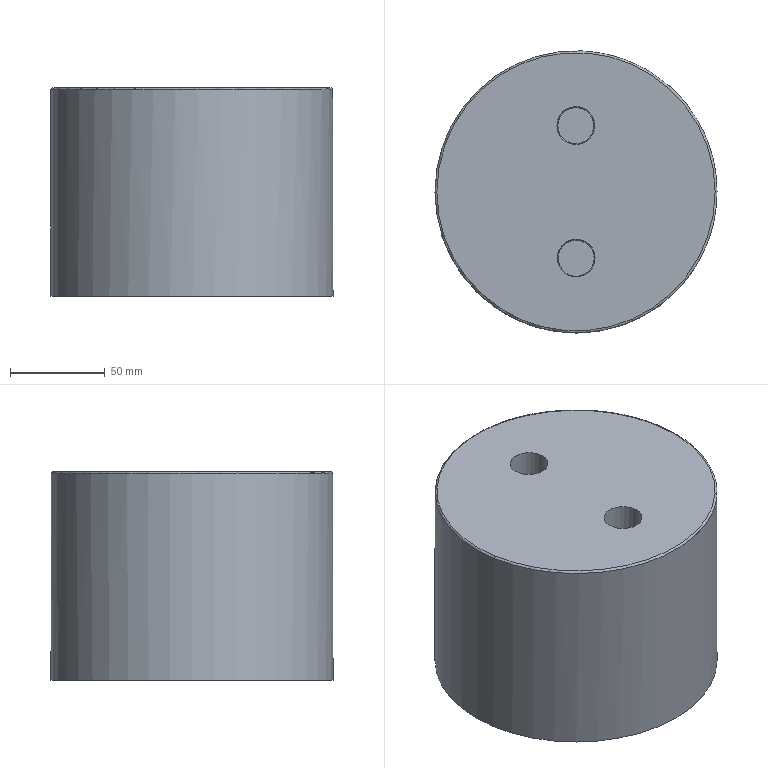Component | NX | A_PART_8 | 1 solid | 16 faces | box 149 x 149 x 110 mm | volume 1872912 mm3 | plane 8 | cylinder 5 | torus 3 | commonest cylinder face diameters 20 x2 149 x1 60 x1 15 x1
STEP:
#1=CARTESIAN_POINT('',(0.,0.,0.));
#2=DIRECTION('',(0.,0.,1.));
#3=DIRECTION('',(1.,0.,0.));
#4=AXIS2_PLACEMENT_3D('',#1,#2,#3);
#5=CARTESIAN_POINT('',(78.417,257.073,11.984));
#6=VERTEX_POINT('',#5);
#7=CARTESIAN_POINT('',(152.917,257.26,11.984));
#8=DIRECTION('',(0.,0.,-1.));
#9=DIRECTION('',(-1.,-0.0025,0.));
#10=AXIS2_PLACEMENT_3D('',#7,#8,#9);
#11=CIRCLE('',#10,74.5);
#12=CARTESIAN_POINT('',(152.917,257.26,12.984));
#13=DIRECTION('',(0.,0.,-1.));
#14=DIRECTION('',(-1.,-0.0025,0.));
#15=AXIS2_PLACEMENT_3D('',#12,#13,#14);
#16=CYLINDRICAL_SURFACE('',#15,74.5);
#17=CARTESIAN_POINT('',(0.,1.));
#18=DIRECTION('',(1.,0.));
#19=VECTOR('',#18,1.);
#20=LINE('',#17,#19);
#21=(GEOMETRIC_REPRESENTATION_CONTEXT(2)PARAMETRIC_REPRESENTATION_CONTEXT()REPRESENTATION_CONTEXT('',''));
#22=DEFINITIONAL_REPRESENTATION('',(#20),#21);
#23=PCURVE('',#16,#22);
#24=CARTESIAN_POINT('',(152.917,257.26,11.984));
#25=DIRECTION('',(0.,0.,-1.));
#26=DIRECTION('',(-1.,-0.0025,0.));
#27=AXIS2_PLACEMENT_3D('',#24,#25,#26);
#28=TOROIDAL_SURFACE('',#27,73.5,1.);
#29=CARTESIAN_POINT('',(0.,6.283));
#30=DIRECTION('',(1.,0.));
#31=VECTOR('',#30,1.);
#32=LINE('',#29,#31);
#33=(GEOMETRIC_REPRESENTATION_CONTEXT(2)PARAMETRIC_REPRESENTATION_CONTEXT()REPRESENTATION_CONTEXT('',''));
#34=DEFINITIONAL_REPRESENTATION('',(#32),#33);
#35=PCURVE('',#28,#34);
#36=SURFACE_CURVE('',#11,(#23,#35),.PCURVE_S1.);
#37=EDGE_CURVE('',#6,#6,#36,.T.);
#38=ORIENTED_EDGE('',*,*,#37,.T.);
#39=CARTESIAN_POINT('',(78.417,257.073,-97.016));
#40=VERTEX_POINT('',#39);
#41=CARTESIAN_POINT('',(78.417,257.073,11.984));
#42=CARTESIAN_POINT('',(78.417,257.073,-97.016));
#43=B_SPLINE_CURVE_WITH_KNOTS('',1,(#41,#42),.UNSPECIFIED.,.F.,.F.,(2,2),(1.,110.),.PIECEWISE_BEZIER_KNOTS.);
#44=CARTESIAN_POINT('',(6.283,0.));
#45=DIRECTION('',(0.,1.));
#46=VECTOR('',#45,1.);
#47=LINE('',#44,#46);
#48=(GEOMETRIC_REPRESENTATION_CONTEXT(2)PARAMETRIC_REPRESENTATION_CONTEXT()REPRESENTATION_CONTEXT('',''));
#49=DEFINITIONAL_REPRESENTATION('',(#47),#48);
#50=PCURVE('',#16,#49);
#51=CARTESIAN_POINT('',(0.,0.));
#52=DIRECTION('',(0.,1.));
#53=VECTOR('',#52,1.);
#54=LINE('',#51,#53);
#55=(GEOMETRIC_REPRESENTATION_CONTEXT(2)PARAMETRIC_REPRESENTATION_CONTEXT()REPRESENTATION_CONTEXT('',''));
#56=DEFINITIONAL_REPRESENTATION('',(#54),#55);
#57=PCURVE('',#16,#56);
#58=SEAM_CURVE('',#43,(#50,#57),.PCURVE_S1.);
#59=EDGE_CURVE('',#6,#40,#58,.T.);
#60=ORIENTED_EDGE('',*,*,#59,.T.);
#61=CARTESIAN_POINT('',(227.417,257.446,-97.016));
#62=VERTEX_POINT('',#61);
#63=CARTESIAN_POINT('',(152.917,257.26,-97.016));
#64=DIRECTION('',(0.,0.,-1.));
#65=DIRECTION('',(1.,0.0025,0.));
#66=AXIS2_PLACEMENT_3D('',#63,#64,#65);
#67=CIRCLE('',#66,74.5);
#68=CARTESIAN_POINT('',(3.142,110.));
#69=DIRECTION('',(1.,0.));
#70=VECTOR('',#69,1.);
#71=LINE('',#68,#70);
#72=(GEOMETRIC_REPRESENTATION_CONTEXT(2)PARAMETRIC_REPRESENTATION_CONTEXT()REPRESENTATION_CONTEXT('',''));
#73=DEFINITIONAL_REPRESENTATION('',(#71),#72);
#74=PCURVE('',#16,#73);
#75=CARTESIAN_POINT('',(152.917,257.26,-97.016));
#76=DIRECTION('',(0.,0.,-1.));
#77=DIRECTION('',(-1.,-0.0025,0.));
#78=AXIS2_PLACEMENT_3D('',#75,#76,#77);
#79=PLANE('',#78);
#80=CARTESIAN_POINT('',(0.,0.));
#81=DIRECTION('',(-1.,0.));
#82=AXIS2_PLACEMENT_2D('',#80,#81);
#83=CIRCLE('',#82,74.5);
#84=(GEOMETRIC_REPRESENTATION_CONTEXT(2)PARAMETRIC_REPRESENTATION_CONTEXT()REPRESENTATION_CONTEXT('',''));
#85=DEFINITIONAL_REPRESENTATION('',(#83),#84);
#86=PCURVE('',#79,#85);
#87=SURFACE_CURVE('',#67,(#74,#86),.PCURVE_S1.);
#88=EDGE_CURVE('',#62,#40,#87,.T.);
#89=ORIENTED_EDGE('',*,*,#88,.F.);
#90=CARTESIAN_POINT('',(152.917,257.26,-97.016));
#91=DIRECTION('',(0.,0.,-1.));
#92=DIRECTION('',(1.,0.0025,0.));
#93=AXIS2_PLACEMENT_3D('',#90,#91,#92);
#94=CIRCLE('',#93,74.5);
#95=CARTESIAN_POINT('',(-3.142,110.));
#96=DIRECTION('',(1.,0.));
#97=VECTOR('',#96,1.);
#98=LINE('',#95,#97);
#99=(GEOMETRIC_REPRESENTATION_CONTEXT(2)PARAMETRIC_REPRESENTATION_CONTEXT()REPRESENTATION_CONTEXT('',''));
#100=DEFINITIONAL_REPRESENTATION('',(#98),#99);
#101=PCURVE('',#16,#100);
#102=CARTESIAN_POINT('',(0.,0.));
#103=DIRECTION('',(-1.,0.));
#104=AXIS2_PLACEMENT_2D('',#102,#103);
#105=CIRCLE('',#104,74.5);
#106=(GEOMETRIC_REPRESENTATION_CONTEXT(2)PARAMETRIC_REPRESENTATION_CONTEXT()REPRESENTATION_CONTEXT('',''));
#107=DEFINITIONAL_REPRESENTATION('',(#105),#106);
#108=PCURVE('',#79,#107);
#109=SURFACE_CURVE('',#94,(#101,#108),.PCURVE_S1.);
#110=EDGE_CURVE('',#40,#62,#109,.T.);
#111=ORIENTED_EDGE('',*,*,#110,.F.);
#112=ORIENTED_EDGE('',*,*,#59,.F.);
#113=EDGE_LOOP('',(#38,#60,#89,#111,#112));
#114=FACE_BOUND('',#113,.T.);
#115=ADVANCED_FACE('',(#114),#16,.T.);
#116=CARTESIAN_POINT('',(163.004,222.285,12.984));
#117=VERTEX_POINT('',#116);
#118=CARTESIAN_POINT('',(153.004,222.26,12.984));
#119=DIRECTION('',(0.,0.,-1.));
#120=DIRECTION('',(1.,0.0025,0.));
#121=AXIS2_PLACEMENT_3D('',#118,#119,#120);
#122=CIRCLE('',#121,10.);
#123=CARTESIAN_POINT('',(152.917,257.26,12.984));
#124=DIRECTION('',(0.,0.,-1.));
#125=DIRECTION('',(-1.,-0.0025,0.));
#126=AXIS2_PLACEMENT_3D('',#123,#124,#125);
#127=PLANE('',#126);
#128=CARTESIAN_POINT('',(0.,-35.));
#129=DIRECTION('',(-1.,0.));
#130=AXIS2_PLACEMENT_2D('',#128,#129);
#131=CIRCLE('',#130,10.);
#132=(GEOMETRIC_REPRESENTATION_CONTEXT(2)PARAMETRIC_REPRESENTATION_CONTEXT()REPRESENTATION_CONTEXT('',''));
#133=DEFINITIONAL_REPRESENTATION('',(#131),#132);
#134=PCURVE('',#127,#133);
#135=CARTESIAN_POINT('',(153.004,222.26,-42.016));
#136=DIRECTION('',(0.,0.,1.));
#137=DIRECTION('',(1.,0.0025,0.));
#138=AXIS2_PLACEMENT_3D('',#135,#136,#137);
#139=CYLINDRICAL_SURFACE('',#138,10.);
#140=CARTESIAN_POINT('',(6.283,55.));
#141=DIRECTION('',(-1.,0.));
#142=VECTOR('',#141,1.);
#143=LINE('',#140,#142);
#144=(GEOMETRIC_REPRESENTATION_CONTEXT(2)PARAMETRIC_REPRESENTATION_CONTEXT()REPRESENTATION_CONTEXT('',''));
#145=DEFINITIONAL_REPRESENTATION('',(#143),#144);
#146=PCURVE('',#139,#145);
#147=SURFACE_CURVE('',#122,(#134,#146),.PCURVE_S1.);
#148=EDGE_CURVE('',#117,#117,#147,.T.);
#149=ORIENTED_EDGE('',*,*,#148,.T.);
#150=EDGE_LOOP('',(#149));
#151=FACE_BOUND('',#150,.T.);
#152=CARTESIAN_POINT('',(162.829,292.285,12.984));
#153=VERTEX_POINT('',#152);
#154=CARTESIAN_POINT('',(152.829,292.26,12.984));
#155=DIRECTION('',(0.,0.,-1.));
#156=DIRECTION('',(1.,0.0025,0.));
#157=AXIS2_PLACEMENT_3D('',#154,#155,#156);
#158=CIRCLE('',#157,10.);
#159=CARTESIAN_POINT('',(0.,35.));
#160=DIRECTION('',(-1.,0.));
#161=AXIS2_PLACEMENT_2D('',#159,#160);
#162=CIRCLE('',#161,10.);
#163=(GEOMETRIC_REPRESENTATION_CONTEXT(2)PARAMETRIC_REPRESENTATION_CONTEXT()REPRESENTATION_CONTEXT('',''));
#164=DEFINITIONAL_REPRESENTATION('',(#162),#163);
#165=PCURVE('',#127,#164);
#166=CARTESIAN_POINT('',(152.829,292.26,-42.016));
#167=DIRECTION('',(0.,0.,1.));
#168=DIRECTION('',(1.,0.0025,0.));
#169=AXIS2_PLACEMENT_3D('',#166,#167,#168);
#170=CYLINDRICAL_SURFACE('',#169,10.);
#171=CARTESIAN_POINT('',(6.283,55.));
#172=DIRECTION('',(-1.,0.));
#173=VECTOR('',#172,1.);
#174=LINE('',#171,#173);
#175=(GEOMETRIC_REPRESENTATION_CONTEXT(2)PARAMETRIC_REPRESENTATION_CONTEXT()REPRESENTATION_CONTEXT('',''));
#176=DEFINITIONAL_REPRESENTATION('',(#174),#175);
#177=PCURVE('',#170,#176);
#178=SURFACE_CURVE('',#158,(#165,#177),.PCURVE_S1.);
#179=EDGE_CURVE('',#153,#153,#178,.T.);
#180=ORIENTED_EDGE('',*,*,#179,.T.);
#181=EDGE_LOOP('',(#180));
#182=FACE_BOUND('',#181,.T.);
#183=CARTESIAN_POINT('',(79.417,257.076,12.984));
#184=VERTEX_POINT('',#183);
#185=CARTESIAN_POINT('',(152.917,257.26,12.984));
#186=DIRECTION('',(0.,0.,1.));
#187=DIRECTION('',(-1.,-0.0025,0.));
#188=AXIS2_PLACEMENT_3D('',#185,#186,#187);
#189=CIRCLE('',#188,73.5);
#190=CARTESIAN_POINT('',(73.5,-0.));
#191=CARTESIAN_POINT('',(73.5,-127.306));
#192=CARTESIAN_POINT('',(-36.75,-63.653));
#193=CARTESIAN_POINT('',(-147.,0.));
#194=CARTESIAN_POINT('',(-36.75,63.653));
#195=CARTESIAN_POINT('',(73.5,127.306));
#196=CARTESIAN_POINT('',(73.5,-0.));
#197=(BOUNDED_CURVE()B_SPLINE_CURVE(2,(#190,#191,#192,#193,#194,#195,#196),.UNSPECIFIED.,.T.,.F.)B_SPLINE_CURVE_WITH_KNOTS((1,2,2,2,2,1),(-2.094,0.,2.094,4.189,6.283,8.378),.UNSPECIFIED.)CURVE()GEOMETRIC_REPRESENTATION_ITEM()RATIONAL_B_SPLINE_CURVE((1.,0.5,1.,0.5,1.,0.5,1.))REPRESENTATION_ITEM(''));
#198=(GEOMETRIC_REPRESENTATION_CONTEXT(2)PARAMETRIC_REPRESENTATION_CONTEXT()REPRESENTATION_CONTEXT('',''));
#199=DEFINITIONAL_REPRESENTATION('',(#197),#198);
#200=PCURVE('',#127,#199);
#201=CARTESIAN_POINT('',(6.283,4.712));
#202=DIRECTION('',(-1.,0.));
#203=VECTOR('',#202,1.);
#204=LINE('',#201,#203);
#205=(GEOMETRIC_REPRESENTATION_CONTEXT(2)PARAMETRIC_REPRESENTATION_CONTEXT()REPRESENTATION_CONTEXT('',''));
#206=DEFINITIONAL_REPRESENTATION('',(#204),#205);
#207=PCURVE('',#28,#206);
#208=SURFACE_CURVE('',#189,(#200,#207),.PCURVE_S1.);
#209=EDGE_CURVE('',#184,#184,#208,.T.);
#210=ORIENTED_EDGE('',*,*,#209,.T.);
#211=EDGE_LOOP('',(#210));
#212=FACE_BOUND('',#211,.T.);
#213=ADVANCED_FACE('',(#151,#182,#212),#127,.F.);
#214=CARTESIAN_POINT('',(182.917,257.335,-97.016));
#215=VERTEX_POINT('',#214);
#216=CARTESIAN_POINT('',(152.917,257.26,-97.016));
#217=DIRECTION('',(0.,0.,-1.));
#218=DIRECTION('',(1.,0.0025,0.));
#219=AXIS2_PLACEMENT_3D('',#216,#217,#218);
#220=CIRCLE('',#219,30.);
#221=CARTESIAN_POINT('',(0.,0.));
#222=DIRECTION('',(-1.,0.));
#223=AXIS2_PLACEMENT_2D('',#221,#222);
#224=CIRCLE('',#223,30.);
#225=(GEOMETRIC_REPRESENTATION_CONTEXT(2)PARAMETRIC_REPRESENTATION_CONTEXT()REPRESENTATION_CONTEXT('',''));
#226=DEFINITIONAL_REPRESENTATION('',(#224),#225);
#227=PCURVE('',#79,#226);
#228=CARTESIAN_POINT('',(152.917,257.26,-95.016));
#229=DIRECTION('',(0.,0.,-1.));
#230=DIRECTION('',(-1.,-0.0025,0.));
#231=AXIS2_PLACEMENT_3D('',#228,#229,#230);
#232=CYLINDRICAL_SURFACE('',#231,30.);
#233=CARTESIAN_POINT('',(3.142,2.));
#234=DIRECTION('',(1.,0.));
#235=VECTOR('',#234,1.);
#236=LINE('',#233,#235);
#237=(GEOMETRIC_REPRESENTATION_CONTEXT(2)PARAMETRIC_REPRESENTATION_CONTEXT()REPRESENTATION_CONTEXT('',''));
#238=DEFINITIONAL_REPRESENTATION('',(#236),#237);
#239=PCURVE('',#232,#238);
#240=SURFACE_CURVE('',#220,(#227,#239),.PCURVE_S1.);
#241=EDGE_CURVE('',#215,#215,#240,.T.);
#242=ORIENTED_EDGE('',*,*,#241,.F.);
#243=EDGE_LOOP('',(#242));
#244=FACE_BOUND('',#243,.T.);
#245=ORIENTED_EDGE('',*,*,#88,.T.);
#246=ORIENTED_EDGE('',*,*,#110,.T.);
#247=EDGE_LOOP('',(#245,#246));
#248=FACE_BOUND('',#247,.T.);
#249=ADVANCED_FACE('',(#244,#248),#79,.T.);
#250=ORIENTED_EDGE('',*,*,#209,.F.);
#251=CARTESIAN_POINT('',(79.417,257.076,12.984));
#252=CARTESIAN_POINT('',(79.15,257.075,12.984));
#253=CARTESIAN_POINT('',(78.889,257.075,12.899));
#254=CARTESIAN_POINT('',(78.665,257.074,12.736));
#255=CARTESIAN_POINT('',(78.502,257.074,12.511));
#256=CARTESIAN_POINT('',(78.417,257.073,12.251));
#257=CARTESIAN_POINT('',(78.417,257.073,11.984));
#258=(BOUNDED_CURVE()B_SPLINE_CURVE(6,(#251,#252,#253,#254,#255,#256,#257),.UNSPECIFIED.,.F.,.F.)B_SPLINE_CURVE_WITH_KNOTS((7,7),(4.712,6.283),.PIECEWISE_BEZIER_KNOTS.)CURVE()GEOMETRIC_REPRESENTATION_ITEM()RATIONAL_B_SPLINE_CURVE((1.031,1.01,0.9979,0.994,0.9979,1.01,1.031))REPRESENTATION_ITEM(''));
#259=CARTESIAN_POINT('',(6.283,0.));
#260=DIRECTION('',(0.,1.));
#261=VECTOR('',#260,1.);
#262=LINE('',#259,#261);
#263=(GEOMETRIC_REPRESENTATION_CONTEXT(2)PARAMETRIC_REPRESENTATION_CONTEXT()REPRESENTATION_CONTEXT('',''));
#264=DEFINITIONAL_REPRESENTATION('',(#262),#263);
#265=PCURVE('',#28,#264);
#266=CARTESIAN_POINT('',(0.,0.));
#267=DIRECTION('',(0.,1.));
#268=VECTOR('',#267,1.);
#269=LINE('',#266,#268);
#270=(GEOMETRIC_REPRESENTATION_CONTEXT(2)PARAMETRIC_REPRESENTATION_CONTEXT()REPRESENTATION_CONTEXT('',''));
#271=DEFINITIONAL_REPRESENTATION('',(#269),#270);
#272=PCURVE('',#28,#271);
#273=SEAM_CURVE('',#258,(#265,#272),.PCURVE_S1.);
#274=EDGE_CURVE('',#184,#6,#273,.T.);
#275=ORIENTED_EDGE('',*,*,#274,.T.);
#276=ORIENTED_EDGE('',*,*,#37,.F.);
#277=ORIENTED_EDGE('',*,*,#274,.F.);
#278=EDGE_LOOP('',(#250,#275,#276,#277));
#279=FACE_BOUND('',#278,.T.);
#280=ADVANCED_FACE('',(#279),#28,.T.);
#281=CARTESIAN_POINT('',(162.829,292.285,-41.516));
#282=VERTEX_POINT('',#281);
#283=CARTESIAN_POINT('',(142.829,292.235,-41.516));
#284=VERTEX_POINT('',#283);
#285=CARTESIAN_POINT('',(152.829,292.26,-41.516));
#286=DIRECTION('',(0.,0.,-1.));
#287=DIRECTION('',(-1.,-0.0025,0.));
#288=AXIS2_PLACEMENT_3D('',#285,#286,#287);
#289=CIRCLE('',#288,10.);
#290=CARTESIAN_POINT('',(9.425,0.5));
#291=DIRECTION('',(-1.,0.));
#292=VECTOR('',#291,1.);
#293=LINE('',#290,#292);
#294=(GEOMETRIC_REPRESENTATION_CONTEXT(2)PARAMETRIC_REPRESENTATION_CONTEXT()REPRESENTATION_CONTEXT('',''));
#295=DEFINITIONAL_REPRESENTATION('',(#293),#294);
#296=PCURVE('',#170,#295);
#297=CARTESIAN_POINT('',(152.829,292.26,-41.516));
#298=DIRECTION('',(0.,0.,-1.));
#299=DIRECTION('',(-1.,-0.0025,0.));
#300=AXIS2_PLACEMENT_3D('',#297,#298,#299);
#301=TOROIDAL_SURFACE('',#300,9.5,0.5);
#302=CARTESIAN_POINT('',(0.,6.283));
#303=DIRECTION('',(1.,0.));
#304=VECTOR('',#303,1.);
#305=LINE('',#302,#304);
#306=(GEOMETRIC_REPRESENTATION_CONTEXT(2)PARAMETRIC_REPRESENTATION_CONTEXT()REPRESENTATION_CONTEXT('',''));
#307=DEFINITIONAL_REPRESENTATION('',(#305),#306);
#308=PCURVE('',#301,#307);
#309=SURFACE_CURVE('',#289,(#296,#308),.PCURVE_S1.);
#310=EDGE_CURVE('',#282,#284,#309,.T.);
#311=ORIENTED_EDGE('',*,*,#310,.F.);
#312=CARTESIAN_POINT('',(162.829,292.285,-41.516));
#313=CARTESIAN_POINT('',(162.829,292.285,12.984));
#314=B_SPLINE_CURVE_WITH_KNOTS('',1,(#312,#313),.UNSPECIFIED.,.F.,.F.,(2,2),(0.5,55.),.PIECEWISE_BEZIER_KNOTS.);
#315=CARTESIAN_POINT('',(6.283,0.));
#316=DIRECTION('',(0.,1.));
#317=VECTOR('',#316,1.);
#318=LINE('',#315,#317);
#319=(GEOMETRIC_REPRESENTATION_CONTEXT(2)PARAMETRIC_REPRESENTATION_CONTEXT()REPRESENTATION_CONTEXT('',''));
#320=DEFINITIONAL_REPRESENTATION('',(#318),#319);
#321=PCURVE('',#170,#320);
#322=CARTESIAN_POINT('',(0.,0.));
#323=DIRECTION('',(0.,1.));
#324=VECTOR('',#323,1.);
#325=LINE('',#322,#324);
#326=(GEOMETRIC_REPRESENTATION_CONTEXT(2)PARAMETRIC_REPRESENTATION_CONTEXT()REPRESENTATION_CONTEXT('',''));
#327=DEFINITIONAL_REPRESENTATION('',(#325),#326);
#328=PCURVE('',#170,#327);
#329=SEAM_CURVE('',#314,(#321,#328),.PCURVE_S1.);
#330=EDGE_CURVE('',#282,#153,#329,.T.);
#331=ORIENTED_EDGE('',*,*,#330,.T.);
#332=ORIENTED_EDGE('',*,*,#179,.T.);
#333=ORIENTED_EDGE('',*,*,#330,.F.);
#334=CARTESIAN_POINT('',(152.829,292.26,-41.516));
#335=DIRECTION('',(0.,0.,-1.));
#336=DIRECTION('',(-1.,-0.0025,0.));
#337=AXIS2_PLACEMENT_3D('',#334,#335,#336);
#338=CIRCLE('',#337,10.);
#339=CARTESIAN_POINT('',(3.142,0.5));
#340=DIRECTION('',(-1.,0.));
#341=VECTOR('',#340,1.);
#342=LINE('',#339,#341);
#343=(GEOMETRIC_REPRESENTATION_CONTEXT(2)PARAMETRIC_REPRESENTATION_CONTEXT()REPRESENTATION_CONTEXT('',''));
#344=DEFINITIONAL_REPRESENTATION('',(#342),#343);
#345=PCURVE('',#170,#344);
#346=CARTESIAN_POINT('',(0.,6.283));
#347=DIRECTION('',(1.,0.));
#348=VECTOR('',#347,1.);
#349=LINE('',#346,#348);
#350=(GEOMETRIC_REPRESENTATION_CONTEXT(2)PARAMETRIC_REPRESENTATION_CONTEXT()REPRESENTATION_CONTEXT('',''));
#351=DEFINITIONAL_REPRESENTATION('',(#349),#350);
#352=PCURVE('',#301,#351);
#353=SURFACE_CURVE('',#338,(#345,#352),.PCURVE_S1.);
#354=EDGE_CURVE('',#284,#282,#353,.T.);
#355=ORIENTED_EDGE('',*,*,#354,.F.);
#356=EDGE_LOOP('',(#311,#331,#332,#333,#355));
#357=FACE_BOUND('',#356,.F.);
#358=ADVANCED_FACE('',(#357),#170,.F.);
#359=CARTESIAN_POINT('',(143.329,292.236,-42.016));
#360=VERTEX_POINT('',#359);
#361=CARTESIAN_POINT('',(152.829,292.26,-42.016));
#362=DIRECTION('',(0.,0.,1.));
#363=DIRECTION('',(-1.,-0.0025,0.));
#364=AXIS2_PLACEMENT_3D('',#361,#362,#363);
#365=CIRCLE('',#364,9.5);
#366=CARTESIAN_POINT('',(152.829,292.26,-42.016));
#367=DIRECTION('',(0.,0.,-1.));
#368=DIRECTION('',(-1.,-0.0025,0.));
#369=AXIS2_PLACEMENT_3D('',#366,#367,#368);
#370=PLANE('',#369);
#371=CARTESIAN_POINT('',(9.5,-0.));
#372=CARTESIAN_POINT('',(9.5,-16.454));
#373=CARTESIAN_POINT('',(-4.75,-8.227));
#374=CARTESIAN_POINT('',(-19.,0.));
#375=CARTESIAN_POINT('',(-4.75,8.227));
#376=CARTESIAN_POINT('',(9.5,16.454));
#377=CARTESIAN_POINT('',(9.5,-0.));
#378=(BOUNDED_CURVE()B_SPLINE_CURVE(2,(#371,#372,#373,#374,#375,#376,#377),.UNSPECIFIED.,.T.,.F.)B_SPLINE_CURVE_WITH_KNOTS((1,2,2,2,2,1),(-2.094,0.,2.094,4.189,6.283,8.378),.UNSPECIFIED.)CURVE()GEOMETRIC_REPRESENTATION_ITEM()RATIONAL_B_SPLINE_CURVE((1.,0.5,1.,0.5,1.,0.5,1.))REPRESENTATION_ITEM(''));
#379=(GEOMETRIC_REPRESENTATION_CONTEXT(2)PARAMETRIC_REPRESENTATION_CONTEXT()REPRESENTATION_CONTEXT('',''));
#380=DEFINITIONAL_REPRESENTATION('',(#378),#379);
#381=PCURVE('',#370,#380);
#382=CARTESIAN_POINT('',(6.283,7.854));
#383=DIRECTION('',(-1.,0.));
#384=VECTOR('',#383,1.);
#385=LINE('',#382,#384);
#386=(GEOMETRIC_REPRESENTATION_CONTEXT(2)PARAMETRIC_REPRESENTATION_CONTEXT()REPRESENTATION_CONTEXT('',''));
#387=DEFINITIONAL_REPRESENTATION('',(#385),#386);
#388=PCURVE('',#301,#387);
#389=SURFACE_CURVE('',#365,(#381,#388),.PCURVE_S1.);
#390=EDGE_CURVE('',#360,#360,#389,.T.);
#391=ORIENTED_EDGE('',*,*,#390,.T.);
#392=EDGE_LOOP('',(#391));
#393=FACE_BOUND('',#392,.T.);
#394=ADVANCED_FACE('',(#393),#370,.F.);
#395=CARTESIAN_POINT('',(163.004,222.285,-41.516));
#396=VERTEX_POINT('',#395);
#397=CARTESIAN_POINT('',(143.004,222.235,-41.516));
#398=VERTEX_POINT('',#397);
#399=CARTESIAN_POINT('',(153.004,222.26,-41.516));
#400=DIRECTION('',(0.,0.,-1.));
#401=DIRECTION('',(-1.,-0.0025,0.));
#402=AXIS2_PLACEMENT_3D('',#399,#400,#401);
#403=CIRCLE('',#402,10.);
#404=CARTESIAN_POINT('',(9.425,0.5));
#405=DIRECTION('',(-1.,0.));
#406=VECTOR('',#405,1.);
#407=LINE('',#404,#406);
#408=(GEOMETRIC_REPRESENTATION_CONTEXT(2)PARAMETRIC_REPRESENTATION_CONTEXT()REPRESENTATION_CONTEXT('',''));
#409=DEFINITIONAL_REPRESENTATION('',(#407),#408);
#410=PCURVE('',#139,#409);
#411=CARTESIAN_POINT('',(153.004,222.26,-41.516));
#412=DIRECTION('',(0.,0.,-1.));
#413=DIRECTION('',(-1.,-0.0025,0.));
#414=AXIS2_PLACEMENT_3D('',#411,#412,#413);
#415=TOROIDAL_SURFACE('',#414,9.5,0.5);
#416=CARTESIAN_POINT('',(-0.,6.283));
#417=DIRECTION('',(1.,0.));
#418=VECTOR('',#417,1.);
#419=LINE('',#416,#418);
#420=(GEOMETRIC_REPRESENTATION_CONTEXT(2)PARAMETRIC_REPRESENTATION_CONTEXT()REPRESENTATION_CONTEXT('',''));
#421=DEFINITIONAL_REPRESENTATION('',(#419),#420);
#422=PCURVE('',#415,#421);
#423=SURFACE_CURVE('',#403,(#410,#422),.PCURVE_S1.);
#424=EDGE_CURVE('',#396,#398,#423,.T.);
#425=ORIENTED_EDGE('',*,*,#424,.F.);
#426=CARTESIAN_POINT('',(163.004,222.285,-41.516));
#427=CARTESIAN_POINT('',(163.004,222.285,12.984));
#428=B_SPLINE_CURVE_WITH_KNOTS('',1,(#426,#427),.UNSPECIFIED.,.F.,.F.,(2,2),(0.5,55.),.PIECEWISE_BEZIER_KNOTS.);
#429=CARTESIAN_POINT('',(6.283,0.));
#430=DIRECTION('',(0.,1.));
#431=VECTOR('',#430,1.);
#432=LINE('',#429,#431);
#433=(GEOMETRIC_REPRESENTATION_CONTEXT(2)PARAMETRIC_REPRESENTATION_CONTEXT()REPRESENTATION_CONTEXT('',''));
#434=DEFINITIONAL_REPRESENTATION('',(#432),#433);
#435=PCURVE('',#139,#434);
#436=CARTESIAN_POINT('',(0.,0.));
#437=DIRECTION('',(0.,1.));
#438=VECTOR('',#437,1.);
#439=LINE('',#436,#438);
#440=(GEOMETRIC_REPRESENTATION_CONTEXT(2)PARAMETRIC_REPRESENTATION_CONTEXT()REPRESENTATION_CONTEXT('',''));
#441=DEFINITIONAL_REPRESENTATION('',(#439),#440);
#442=PCURVE('',#139,#441);
#443=SEAM_CURVE('',#428,(#435,#442),.PCURVE_S1.);
#444=EDGE_CURVE('',#396,#117,#443,.T.);
#445=ORIENTED_EDGE('',*,*,#444,.T.);
#446=ORIENTED_EDGE('',*,*,#148,.T.);
#447=ORIENTED_EDGE('',*,*,#444,.F.);
#448=CARTESIAN_POINT('',(153.004,222.26,-41.516));
#449=DIRECTION('',(0.,0.,-1.));
#450=DIRECTION('',(-1.,-0.0025,0.));
#451=AXIS2_PLACEMENT_3D('',#448,#449,#450);
#452=CIRCLE('',#451,10.);
#453=CARTESIAN_POINT('',(3.142,0.5));
#454=DIRECTION('',(-1.,0.));
#455=VECTOR('',#454,1.);
#456=LINE('',#453,#455);
#457=(GEOMETRIC_REPRESENTATION_CONTEXT(2)PARAMETRIC_REPRESENTATION_CONTEXT()REPRESENTATION_CONTEXT('',''));
#458=DEFINITIONAL_REPRESENTATION('',(#456),#457);
#459=PCURVE('',#139,#458);
#460=CARTESIAN_POINT('',(0.,6.283));
#461=DIRECTION('',(1.,0.));
#462=VECTOR('',#461,1.);
#463=LINE('',#460,#462);
#464=(GEOMETRIC_REPRESENTATION_CONTEXT(2)PARAMETRIC_REPRESENTATION_CONTEXT()REPRESENTATION_CONTEXT('',''));
#465=DEFINITIONAL_REPRESENTATION('',(#463),#464);
#466=PCURVE('',#415,#465);
#467=SURFACE_CURVE('',#452,(#459,#466),.PCURVE_S1.);
#468=EDGE_CURVE('',#398,#396,#467,.T.);
#469=ORIENTED_EDGE('',*,*,#468,.F.);
#470=EDGE_LOOP('',(#425,#445,#446,#447,#469));
#471=FACE_BOUND('',#470,.F.);
#472=ADVANCED_FACE('',(#471),#139,.F.);
#473=CARTESIAN_POINT('',(143.504,222.236,-42.016));
#474=VERTEX_POINT('',#473);
#475=CARTESIAN_POINT('',(153.004,222.26,-42.016));
#476=DIRECTION('',(0.,0.,1.));
#477=DIRECTION('',(-1.,-0.0025,0.));
#478=AXIS2_PLACEMENT_3D('',#475,#476,#477);
#479=CIRCLE('',#478,9.5);
#480=CARTESIAN_POINT('',(153.004,222.26,-42.016));
#481=DIRECTION('',(0.,0.,-1.));
#482=DIRECTION('',(-1.,-0.0025,0.));
#483=AXIS2_PLACEMENT_3D('',#480,#481,#482);
#484=PLANE('',#483);
#485=CARTESIAN_POINT('',(9.5,-0.));
#486=CARTESIAN_POINT('',(9.5,-16.454));
#487=CARTESIAN_POINT('',(-4.75,-8.227));
#488=CARTESIAN_POINT('',(-19.,0.));
#489=CARTESIAN_POINT('',(-4.75,8.227));
#490=CARTESIAN_POINT('',(9.5,16.454));
#491=CARTESIAN_POINT('',(9.5,-0.));
#492=(BOUNDED_CURVE()B_SPLINE_CURVE(2,(#485,#486,#487,#488,#489,#490,#491),.UNSPECIFIED.,.T.,.F.)B_SPLINE_CURVE_WITH_KNOTS((1,2,2,2,2,1),(-2.094,0.,2.094,4.189,6.283,8.378),.UNSPECIFIED.)CURVE()GEOMETRIC_REPRESENTATION_ITEM()RATIONAL_B_SPLINE_CURVE((1.,0.5,1.,0.5,1.,0.5,1.))REPRESENTATION_ITEM(''));
#493=(GEOMETRIC_REPRESENTATION_CONTEXT(2)PARAMETRIC_REPRESENTATION_CONTEXT()REPRESENTATION_CONTEXT('',''));
#494=DEFINITIONAL_REPRESENTATION('',(#492),#493);
#495=PCURVE('',#484,#494);
#496=CARTESIAN_POINT('',(6.283,7.854));
#497=DIRECTION('',(-1.,0.));
#498=VECTOR('',#497,1.);
#499=LINE('',#496,#498);
#500=(GEOMETRIC_REPRESENTATION_CONTEXT(2)PARAMETRIC_REPRESENTATION_CONTEXT()REPRESENTATION_CONTEXT('',''));
#501=DEFINITIONAL_REPRESENTATION('',(#499),#500);
#502=PCURVE('',#415,#501);
#503=SURFACE_CURVE('',#479,(#495,#502),.PCURVE_S1.);
#504=EDGE_CURVE('',#474,#474,#503,.T.);
#505=ORIENTED_EDGE('',*,*,#504,.T.);
#506=EDGE_LOOP('',(#505));
#507=FACE_BOUND('',#506,.T.);
#508=ADVANCED_FACE('',(#507),#484,.F.);
#509=ORIENTED_EDGE('',*,*,#310,.T.);
#510=CARTESIAN_POINT('',(142.829,292.235,-41.516));
#511=CARTESIAN_POINT('',(142.829,292.235,-41.65));
#512=CARTESIAN_POINT('',(142.872,292.235,-41.78));
#513=CARTESIAN_POINT('',(142.953,292.235,-41.892));
#514=CARTESIAN_POINT('',(143.065,292.235,-41.974));
#515=CARTESIAN_POINT('',(143.196,292.235,-42.016));
#516=CARTESIAN_POINT('',(143.329,292.236,-42.016));
#517=(BOUNDED_CURVE()B_SPLINE_CURVE(6,(#510,#511,#512,#513,#514,#515,#516),.UNSPECIFIED.,.F.,.F.)B_SPLINE_CURVE_WITH_KNOTS((7,7),(0.,1.571),.PIECEWISE_BEZIER_KNOTS.)CURVE()GEOMETRIC_REPRESENTATION_ITEM()RATIONAL_B_SPLINE_CURVE((1.031,1.01,0.9979,0.994,0.9979,1.01,1.031))REPRESENTATION_ITEM(''));
#518=CARTESIAN_POINT('',(6.283,6.283));
#519=DIRECTION('',(0.,1.));
#520=VECTOR('',#519,1.);
#521=LINE('',#518,#520);
#522=(GEOMETRIC_REPRESENTATION_CONTEXT(2)PARAMETRIC_REPRESENTATION_CONTEXT()REPRESENTATION_CONTEXT('',''));
#523=DEFINITIONAL_REPRESENTATION('',(#521),#522);
#524=PCURVE('',#301,#523);
#525=CARTESIAN_POINT('',(0.,6.283));
#526=DIRECTION('',(0.,1.));
#527=VECTOR('',#526,1.);
#528=LINE('',#525,#527);
#529=(GEOMETRIC_REPRESENTATION_CONTEXT(2)PARAMETRIC_REPRESENTATION_CONTEXT()REPRESENTATION_CONTEXT('',''));
#530=DEFINITIONAL_REPRESENTATION('',(#528),#529);
#531=PCURVE('',#301,#530);
#532=SEAM_CURVE('',#517,(#524,#531),.PCURVE_S1.);
#533=EDGE_CURVE('',#284,#360,#532,.T.);
#534=ORIENTED_EDGE('',*,*,#533,.T.);
#535=ORIENTED_EDGE('',*,*,#390,.T.);
#536=ORIENTED_EDGE('',*,*,#533,.F.);
#537=ORIENTED_EDGE('',*,*,#354,.T.);
#538=EDGE_LOOP('',(#509,#534,#535,#536,#537));
#539=FACE_BOUND('',#538,.F.);
#540=ADVANCED_FACE('',(#539),#301,.F.);
#541=ORIENTED_EDGE('',*,*,#424,.T.);
#542=CARTESIAN_POINT('',(143.004,222.235,-41.516));
#543=CARTESIAN_POINT('',(143.004,222.235,-41.65));
#544=CARTESIAN_POINT('',(143.047,222.235,-41.78));
#545=CARTESIAN_POINT('',(143.128,222.235,-41.892));
#546=CARTESIAN_POINT('',(143.24,222.235,-41.974));
#547=CARTESIAN_POINT('',(143.371,222.236,-42.016));
#548=CARTESIAN_POINT('',(143.504,222.236,-42.016));
#549=(BOUNDED_CURVE()B_SPLINE_CURVE(6,(#542,#543,#544,#545,#546,#547,#548),.UNSPECIFIED.,.F.,.F.)B_SPLINE_CURVE_WITH_KNOTS((7,7),(0.,1.571),.PIECEWISE_BEZIER_KNOTS.)CURVE()GEOMETRIC_REPRESENTATION_ITEM()RATIONAL_B_SPLINE_CURVE((1.031,1.01,0.9979,0.994,0.9979,1.01,1.031))REPRESENTATION_ITEM(''));
#550=CARTESIAN_POINT('',(6.283,6.283));
#551=DIRECTION('',(0.,1.));
#552=VECTOR('',#551,1.);
#553=LINE('',#550,#552);
#554=(GEOMETRIC_REPRESENTATION_CONTEXT(2)PARAMETRIC_REPRESENTATION_CONTEXT()REPRESENTATION_CONTEXT('',''));
#555=DEFINITIONAL_REPRESENTATION('',(#553),#554);
#556=PCURVE('',#415,#555);
#557=CARTESIAN_POINT('',(-0.,6.283));
#558=DIRECTION('',(0.,1.));
#559=VECTOR('',#558,1.);
#560=LINE('',#557,#559);
#561=(GEOMETRIC_REPRESENTATION_CONTEXT(2)PARAMETRIC_REPRESENTATION_CONTEXT()REPRESENTATION_CONTEXT('',''));
#562=DEFINITIONAL_REPRESENTATION('',(#560),#561);
#563=PCURVE('',#415,#562);
#564=SEAM_CURVE('',#549,(#556,#563),.PCURVE_S1.);
#565=EDGE_CURVE('',#398,#474,#564,.T.);
#566=ORIENTED_EDGE('',*,*,#565,.T.);
#567=ORIENTED_EDGE('',*,*,#504,.T.);
#568=ORIENTED_EDGE('',*,*,#565,.F.);
#569=ORIENTED_EDGE('',*,*,#468,.T.);
#570=EDGE_LOOP('',(#541,#566,#567,#568,#569));
#571=FACE_BOUND('',#570,.F.);
#572=ADVANCED_FACE('',(#571),#415,.F.);
#573=CARTESIAN_POINT('',(182.917,257.335,-95.016));
#574=VERTEX_POINT('',#573);
#575=CARTESIAN_POINT('',(152.917,257.26,-95.016));
#576=DIRECTION('',(0.,0.,1.));
#577=DIRECTION('',(1.,0.0025,0.));
#578=AXIS2_PLACEMENT_3D('',#575,#576,#577);
#579=CIRCLE('',#578,30.);
#580=CARTESIAN_POINT('',(9.425,0.));
#581=DIRECTION('',(-1.,0.));
#582=VECTOR('',#581,1.);
#583=LINE('',#580,#582);
#584=(GEOMETRIC_REPRESENTATION_CONTEXT(2)PARAMETRIC_REPRESENTATION_CONTEXT()REPRESENTATION_CONTEXT('',''));
#585=DEFINITIONAL_REPRESENTATION('',(#583),#584);
#586=PCURVE('',#232,#585);
#587=CARTESIAN_POINT('',(152.917,257.26,-95.016));
#588=DIRECTION('',(0.,0.,-1.));
#589=DIRECTION('',(-1.,-0.0025,0.));
#590=AXIS2_PLACEMENT_3D('',#587,#588,#589);
#591=PLANE('',#590);
#592=CARTESIAN_POINT('',(-30.,0.));
#593=CARTESIAN_POINT('',(-30.,51.962));
#594=CARTESIAN_POINT('',(15.,25.981));
#595=CARTESIAN_POINT('',(60.,0.));
#596=CARTESIAN_POINT('',(15.,-25.981));
#597=CARTESIAN_POINT('',(-30.,-51.962));
#598=CARTESIAN_POINT('',(-30.,0.));
#599=(BOUNDED_CURVE()B_SPLINE_CURVE(2,(#592,#593,#594,#595,#596,#597,#598),.UNSPECIFIED.,.T.,.F.)B_SPLINE_CURVE_WITH_KNOTS((1,2,2,2,2,1),(-2.094,0.,2.094,4.189,6.283,8.378),.UNSPECIFIED.)CURVE()GEOMETRIC_REPRESENTATION_ITEM()RATIONAL_B_SPLINE_CURVE((1.,0.5,1.,0.5,1.,0.5,1.))REPRESENTATION_ITEM(''));
#600=(GEOMETRIC_REPRESENTATION_CONTEXT(2)PARAMETRIC_REPRESENTATION_CONTEXT()REPRESENTATION_CONTEXT('',''));
#601=DEFINITIONAL_REPRESENTATION('',(#599),#600);
#602=PCURVE('',#591,#601);
#603=SURFACE_CURVE('',#579,(#586,#602),.PCURVE_S1.);
#604=EDGE_CURVE('',#574,#574,#603,.T.);
#605=ORIENTED_EDGE('',*,*,#604,.F.);
#606=CARTESIAN_POINT('',(182.917,257.335,-95.016));
#607=CARTESIAN_POINT('',(182.917,257.335,-97.016));
#608=B_SPLINE_CURVE_WITH_KNOTS('',1,(#606,#607),.UNSPECIFIED.,.F.,.F.,(2,2),(0.,2.),.PIECEWISE_BEZIER_KNOTS.);
#609=CARTESIAN_POINT('',(9.425,0.));
#610=DIRECTION('',(0.,1.));
#611=VECTOR('',#610,1.);
#612=LINE('',#609,#611);
#613=(GEOMETRIC_REPRESENTATION_CONTEXT(2)PARAMETRIC_REPRESENTATION_CONTEXT()REPRESENTATION_CONTEXT('',''));
#614=DEFINITIONAL_REPRESENTATION('',(#612),#613);
#615=PCURVE('',#232,#614);
#616=CARTESIAN_POINT('',(3.142,0.));
#617=DIRECTION('',(0.,1.));
#618=VECTOR('',#617,1.);
#619=LINE('',#616,#618);
#620=(GEOMETRIC_REPRESENTATION_CONTEXT(2)PARAMETRIC_REPRESENTATION_CONTEXT()REPRESENTATION_CONTEXT('',''));
#621=DEFINITIONAL_REPRESENTATION('',(#619),#620);
#622=PCURVE('',#232,#621);
#623=SEAM_CURVE('',#608,(#615,#622),.PCURVE_S1.);
#624=EDGE_CURVE('',#574,#215,#623,.T.);
#625=ORIENTED_EDGE('',*,*,#624,.T.);
#626=ORIENTED_EDGE('',*,*,#241,.F.);
#627=ORIENTED_EDGE('',*,*,#624,.F.);
#628=EDGE_LOOP('',(#605,#625,#626,#627));
#629=FACE_BOUND('',#628,.F.);
#630=ADVANCED_FACE('',(#629),#232,.F.);
#631=CARTESIAN_POINT('',(145.417,257.241,-95.016));
#632=VERTEX_POINT('',#631);
#633=CARTESIAN_POINT('',(152.917,257.26,-95.016));
#634=DIRECTION('',(0.,0.,-1.));
#635=DIRECTION('',(-1.,-0.0025,0.));
#636=AXIS2_PLACEMENT_3D('',#633,#634,#635);
#637=CIRCLE('',#636,7.5);
#638=CARTESIAN_POINT('',(0.,0.));
#639=DIRECTION('',(1.,0.));
#640=AXIS2_PLACEMENT_2D('',#638,#639);
#641=CIRCLE('',#640,7.5);
#642=(GEOMETRIC_REPRESENTATION_CONTEXT(2)PARAMETRIC_REPRESENTATION_CONTEXT()REPRESENTATION_CONTEXT('',''));
#643=DEFINITIONAL_REPRESENTATION('',(#641),#642);
#644=PCURVE('',#591,#643);
#645=CARTESIAN_POINT('',(152.917,257.26,-64.516));
#646=DIRECTION('',(0.,0.,-1.));
#647=DIRECTION('',(-1.,-0.0025,0.));
#648=AXIS2_PLACEMENT_3D('',#645,#646,#647);
#649=CYLINDRICAL_SURFACE('',#648,7.5);
#650=CARTESIAN_POINT('',(0.,30.5));
#651=DIRECTION('',(1.,0.));
#652=VECTOR('',#651,1.);
#653=LINE('',#650,#652);
#654=(GEOMETRIC_REPRESENTATION_CONTEXT(2)PARAMETRIC_REPRESENTATION_CONTEXT()REPRESENTATION_CONTEXT('',''));
#655=DEFINITIONAL_REPRESENTATION('',(#653),#654);
#656=PCURVE('',#649,#655);
#657=SURFACE_CURVE('',#637,(#644,#656),.PCURVE_S1.);
#658=EDGE_CURVE('',#632,#632,#657,.T.);
#659=ORIENTED_EDGE('',*,*,#658,.F.);
#660=EDGE_LOOP('',(#659));
#661=FACE_BOUND('',#660,.T.);
#662=ORIENTED_EDGE('',*,*,#604,.F.);
#663=EDGE_LOOP('',(#662));
#664=FACE_BOUND('',#663,.T.);
#665=ADVANCED_FACE('',(#661,#664),#591,.T.);
#666=CARTESIAN_POINT('',(145.417,257.241,-64.516));
#667=VERTEX_POINT('',#666);
#668=CARTESIAN_POINT('',(157.432,251.271,-64.516));
#669=VERTEX_POINT('',#668);
#670=CARTESIAN_POINT('',(152.917,257.26,-64.516));
#671=DIRECTION('',(0.,0.,1.));
#672=DIRECTION('',(1.,0.0025,0.));
#673=AXIS2_PLACEMENT_3D('',#670,#671,#672);
#674=CIRCLE('',#673,7.5);
#675=CARTESIAN_POINT('',(9.425,0.));
#676=DIRECTION('',(-1.,0.));
#677=VECTOR('',#676,1.);
#678=LINE('',#675,#677);
#679=(GEOMETRIC_REPRESENTATION_CONTEXT(2)PARAMETRIC_REPRESENTATION_CONTEXT()REPRESENTATION_CONTEXT('',''));
#680=DEFINITIONAL_REPRESENTATION('',(#678),#679);
#681=PCURVE('',#649,#680);
#682=CARTESIAN_POINT('',(152.917,257.26,-64.516));
#683=DIRECTION('',(0.,0.,-1.));
#684=DIRECTION('',(-1.,-0.0025,0.));
#685=AXIS2_PLACEMENT_3D('',#682,#683,#684);
#686=PLANE('',#685);
#687=CARTESIAN_POINT('',(-7.5,0.));
#688=CARTESIAN_POINT('',(-7.5,12.99));
#689=CARTESIAN_POINT('',(3.75,6.495));
#690=CARTESIAN_POINT('',(15.,-0.));
#691=CARTESIAN_POINT('',(3.75,-6.495));
#692=CARTESIAN_POINT('',(-7.5,-12.99));
#693=CARTESIAN_POINT('',(-7.5,0.));
#694=(BOUNDED_CURVE()B_SPLINE_CURVE(2,(#687,#688,#689,#690,#691,#692,#693),.UNSPECIFIED.,.T.,.F.)B_SPLINE_CURVE_WITH_KNOTS((1,2,2,2,2,1),(-2.094,0.,2.094,4.189,6.283,8.378),.UNSPECIFIED.)CURVE()GEOMETRIC_REPRESENTATION_ITEM()RATIONAL_B_SPLINE_CURVE((1.,0.5,1.,0.5,1.,0.5,1.))REPRESENTATION_ITEM(''));
#695=(GEOMETRIC_REPRESENTATION_CONTEXT(2)PARAMETRIC_REPRESENTATION_CONTEXT()REPRESENTATION_CONTEXT('',''));
#696=DEFINITIONAL_REPRESENTATION('',(#694),#695);
#697=PCURVE('',#686,#696);
#698=SURFACE_CURVE('',#674,(#681,#697),.PCURVE_S1.);
#699=EDGE_CURVE('',#667,#669,#698,.T.);
#700=ORIENTED_EDGE('',*,*,#699,.F.);
#701=CARTESIAN_POINT('',(145.417,257.241,-64.516));
#702=CARTESIAN_POINT('',(145.417,257.241,-95.016));
#703=B_SPLINE_CURVE_WITH_KNOTS('',1,(#701,#702),.UNSPECIFIED.,.F.,.F.,(2,2),(0.,30.5),.PIECEWISE_BEZIER_KNOTS.);
#704=CARTESIAN_POINT('',(6.283,0.));
#705=DIRECTION('',(0.,1.));
#706=VECTOR('',#705,1.);
#707=LINE('',#704,#706);
#708=(GEOMETRIC_REPRESENTATION_CONTEXT(2)PARAMETRIC_REPRESENTATION_CONTEXT()REPRESENTATION_CONTEXT('',''));
#709=DEFINITIONAL_REPRESENTATION('',(#707),#708);
#710=PCURVE('',#649,#709);
#711=CARTESIAN_POINT('',(0.,0.));
#712=DIRECTION('',(0.,1.));
#713=VECTOR('',#712,1.);
#714=LINE('',#711,#713);
#715=(GEOMETRIC_REPRESENTATION_CONTEXT(2)PARAMETRIC_REPRESENTATION_CONTEXT()REPRESENTATION_CONTEXT('',''));
#716=DEFINITIONAL_REPRESENTATION('',(#714),#715);
#717=PCURVE('',#649,#716);
#718=SEAM_CURVE('',#703,(#710,#717),.PCURVE_S1.);
#719=EDGE_CURVE('',#667,#632,#718,.T.);
#720=ORIENTED_EDGE('',*,*,#719,.T.);
#721=ORIENTED_EDGE('',*,*,#658,.F.);
#722=ORIENTED_EDGE('',*,*,#719,.F.);
#723=CARTESIAN_POINT('',(157.402,263.271,-64.516));
#724=VERTEX_POINT('',#723);
#725=CARTESIAN_POINT('',(152.917,257.26,-64.516));
#726=DIRECTION('',(0.,0.,1.));
#727=DIRECTION('',(1.,0.0025,0.));
#728=AXIS2_PLACEMENT_3D('',#725,#726,#727);
#729=CIRCLE('',#728,7.5);
#730=CARTESIAN_POINT('',(3.142,0.));
#731=DIRECTION('',(-1.,0.));
#732=VECTOR('',#731,1.);
#733=LINE('',#730,#732);
#734=(GEOMETRIC_REPRESENTATION_CONTEXT(2)PARAMETRIC_REPRESENTATION_CONTEXT()REPRESENTATION_CONTEXT('',''));
#735=DEFINITIONAL_REPRESENTATION('',(#733),#734);
#736=PCURVE('',#649,#735);
#737=CARTESIAN_POINT('',(-7.5,0.));
#738=CARTESIAN_POINT('',(-7.5,12.99));
#739=CARTESIAN_POINT('',(3.75,6.495));
#740=CARTESIAN_POINT('',(15.,-0.));
#741=CARTESIAN_POINT('',(3.75,-6.495));
#742=CARTESIAN_POINT('',(-7.5,-12.99));
#743=CARTESIAN_POINT('',(-7.5,0.));
#744=(BOUNDED_CURVE()B_SPLINE_CURVE(2,(#737,#738,#739,#740,#741,#742,#743),.UNSPECIFIED.,.T.,.F.)B_SPLINE_CURVE_WITH_KNOTS((1,2,2,2,2,1),(-2.094,0.,2.094,4.189,6.283,8.378),.UNSPECIFIED.)CURVE()GEOMETRIC_REPRESENTATION_ITEM()RATIONAL_B_SPLINE_CURVE((1.,0.5,1.,0.5,1.,0.5,1.))REPRESENTATION_ITEM(''));
#745=(GEOMETRIC_REPRESENTATION_CONTEXT(2)PARAMETRIC_REPRESENTATION_CONTEXT()REPRESENTATION_CONTEXT('',''));
#746=DEFINITIONAL_REPRESENTATION('',(#744),#745);
#747=PCURVE('',#686,#746);
#748=SURFACE_CURVE('',#729,(#736,#747),.PCURVE_S1.);
#749=EDGE_CURVE('',#724,#667,#748,.T.);
#750=ORIENTED_EDGE('',*,*,#749,.F.);
#751=CARTESIAN_POINT('',(157.402,263.271,-87.516));
#752=VERTEX_POINT('',#751);
#753=CARTESIAN_POINT('',(157.402,263.271,-64.516));
#754=DIRECTION('',(0.,0.,1.));
#755=VECTOR('',#754,1.);
#756=LINE('',#753,#755);
#757=CARTESIAN_POINT('',(2.214,0.));
#758=DIRECTION('',(0.,-1.));
#759=VECTOR('',#758,1.);
#760=LINE('',#757,#759);
#761=(GEOMETRIC_REPRESENTATION_CONTEXT(2)PARAMETRIC_REPRESENTATION_CONTEXT()REPRESENTATION_CONTEXT('',''));
#762=DEFINITIONAL_REPRESENTATION('',(#760),#761);
#763=PCURVE('',#649,#762);
#764=CARTESIAN_POINT('',(157.402,263.271,-64.516));
#765=DIRECTION('',(1.,0.0025,0.));
#766=DIRECTION('',(-0.0025,1.,0.));
#767=AXIS2_PLACEMENT_3D('',#764,#765,#766);
#768=PLANE('',#767);
#769=CARTESIAN_POINT('',(-0.,0.));
#770=DIRECTION('',(0.,1.));
#771=VECTOR('',#770,1.);
#772=LINE('',#769,#771);
#773=(GEOMETRIC_REPRESENTATION_CONTEXT(2)PARAMETRIC_REPRESENTATION_CONTEXT()REPRESENTATION_CONTEXT('',''));
#774=DEFINITIONAL_REPRESENTATION('',(#772),#773);
#775=PCURVE('',#768,#774);
#776=SURFACE_CURVE('',#756,(#763,#775),.PCURVE_S1.);
#777=EDGE_CURVE('',#752,#724,#776,.T.);
#778=ORIENTED_EDGE('',*,*,#777,.F.);
#779=CARTESIAN_POINT('',(157.432,251.271,-87.516));
#780=VERTEX_POINT('',#779);
#781=CARTESIAN_POINT('',(152.917,257.26,-87.516));
#782=DIRECTION('',(0.,0.,-1.));
#783=DIRECTION('',(1.,0.0025,0.));
#784=AXIS2_PLACEMENT_3D('',#781,#782,#783);
#785=CIRCLE('',#784,7.5);
#786=CARTESIAN_POINT('',(-3.142,23.));
#787=DIRECTION('',(1.,0.));
#788=VECTOR('',#787,1.);
#789=LINE('',#786,#788);
#790=(GEOMETRIC_REPRESENTATION_CONTEXT(2)PARAMETRIC_REPRESENTATION_CONTEXT()REPRESENTATION_CONTEXT('',''));
#791=DEFINITIONAL_REPRESENTATION('',(#789),#790);
#792=PCURVE('',#649,#791);
#793=CARTESIAN_POINT('',(152.917,257.26,-87.516));
#794=DIRECTION('',(0.,0.,1.));
#795=DIRECTION('',(1.,0.0025,0.));
#796=AXIS2_PLACEMENT_3D('',#793,#794,#795);
#797=PLANE('',#796);
#798=CARTESIAN_POINT('',(7.5,-0.));
#799=CARTESIAN_POINT('',(7.5,-12.99));
#800=CARTESIAN_POINT('',(-3.75,-6.495));
#801=CARTESIAN_POINT('',(-15.,0.));
#802=CARTESIAN_POINT('',(-3.75,6.495));
#803=CARTESIAN_POINT('',(7.5,12.99));
#804=CARTESIAN_POINT('',(7.5,-0.));
#805=(BOUNDED_CURVE()B_SPLINE_CURVE(2,(#798,#799,#800,#801,#802,#803,#804),.UNSPECIFIED.,.T.,.F.)B_SPLINE_CURVE_WITH_KNOTS((1,2,2,2,2,1),(-2.094,0.,2.094,4.189,6.283,8.378),.UNSPECIFIED.)CURVE()GEOMETRIC_REPRESENTATION_ITEM()RATIONAL_B_SPLINE_CURVE((1.,0.5,1.,0.5,1.,0.5,1.))REPRESENTATION_ITEM(''));
#806=(GEOMETRIC_REPRESENTATION_CONTEXT(2)PARAMETRIC_REPRESENTATION_CONTEXT()REPRESENTATION_CONTEXT('',''));
#807=DEFINITIONAL_REPRESENTATION('',(#805),#806);
#808=PCURVE('',#797,#807);
#809=SURFACE_CURVE('',#785,(#792,#808),.PCURVE_S1.);
#810=EDGE_CURVE('',#752,#780,#809,.T.);
#811=ORIENTED_EDGE('',*,*,#810,.T.);
#812=CARTESIAN_POINT('',(157.432,251.271,-64.516));
#813=DIRECTION('',(0.,0.,-1.));
#814=VECTOR('',#813,1.);
#815=LINE('',#812,#814);
#816=CARTESIAN_POINT('',(4.069,0.));
#817=DIRECTION('',(0.,1.));
#818=VECTOR('',#817,1.);
#819=LINE('',#816,#818);
#820=(GEOMETRIC_REPRESENTATION_CONTEXT(2)PARAMETRIC_REPRESENTATION_CONTEXT()REPRESENTATION_CONTEXT('',''));
#821=DEFINITIONAL_REPRESENTATION('',(#819),#820);
#822=PCURVE('',#649,#821);
#823=CARTESIAN_POINT('',(-12.,0.));
#824=DIRECTION('',(0.,-1.));
#825=VECTOR('',#824,1.);
#826=LINE('',#823,#825);
#827=(GEOMETRIC_REPRESENTATION_CONTEXT(2)PARAMETRIC_REPRESENTATION_CONTEXT()REPRESENTATION_CONTEXT('',''));
#828=DEFINITIONAL_REPRESENTATION('',(#826),#827);
#829=PCURVE('',#768,#828);
#830=SURFACE_CURVE('',#815,(#822,#829),.PCURVE_S1.);
#831=EDGE_CURVE('',#669,#780,#830,.T.);
#832=ORIENTED_EDGE('',*,*,#831,.F.);
#833=EDGE_LOOP('',(#700,#720,#721,#722,#750,#778,#811,#832));
#834=FACE_BOUND('',#833,.F.);
#835=ADVANCED_FACE('',(#834),#649,.F.);
#836=ORIENTED_EDGE('',*,*,#777,.F.);
#837=CARTESIAN_POINT('',(157.402,263.271,-87.516));
#838=DIRECTION('',(0.0025,-1.,0.));
#839=VECTOR('',#838,1.);
#840=LINE('',#837,#839);
#841=CARTESIAN_POINT('',(0.,-23.));
#842=DIRECTION('',(-1.,0.));
#843=VECTOR('',#842,1.);
#844=LINE('',#841,#843);
#845=(GEOMETRIC_REPRESENTATION_CONTEXT(2)PARAMETRIC_REPRESENTATION_CONTEXT()REPRESENTATION_CONTEXT('',''));
#846=DEFINITIONAL_REPRESENTATION('',(#844),#845);
#847=PCURVE('',#768,#846);
#848=CARTESIAN_POINT('',(4.5,6.));
#849=DIRECTION('',(0.,-1.));
#850=VECTOR('',#849,1.);
#851=LINE('',#848,#850);
#852=(GEOMETRIC_REPRESENTATION_CONTEXT(2)PARAMETRIC_REPRESENTATION_CONTEXT()REPRESENTATION_CONTEXT('',''));
#853=DEFINITIONAL_REPRESENTATION('',(#851),#852);
#854=PCURVE('',#797,#853);
#855=SURFACE_CURVE('',#840,(#847,#854),.PCURVE_S1.);
#856=EDGE_CURVE('',#752,#780,#855,.T.);
#857=ORIENTED_EDGE('',*,*,#856,.T.);
#858=ORIENTED_EDGE('',*,*,#831,.F.);
#859=CARTESIAN_POINT('',(157.402,263.271,-64.516));
#860=DIRECTION('',(-0.0025,1.,0.));
#861=VECTOR('',#860,1.);
#862=LINE('',#859,#861);
#863=CARTESIAN_POINT('',(0.,0.));
#864=DIRECTION('',(1.,0.));
#865=VECTOR('',#864,1.);
#866=LINE('',#863,#865);
#867=(GEOMETRIC_REPRESENTATION_CONTEXT(2)PARAMETRIC_REPRESENTATION_CONTEXT()REPRESENTATION_CONTEXT('',''));
#868=DEFINITIONAL_REPRESENTATION('',(#866),#867);
#869=PCURVE('',#768,#868);
#870=CARTESIAN_POINT('',(-4.5,6.));
#871=DIRECTION('',(0.,1.));
#872=VECTOR('',#871,1.);
#873=LINE('',#870,#872);
#874=(GEOMETRIC_REPRESENTATION_CONTEXT(2)PARAMETRIC_REPRESENTATION_CONTEXT()REPRESENTATION_CONTEXT('',''));
#875=DEFINITIONAL_REPRESENTATION('',(#873),#874);
#876=PCURVE('',#686,#875);
#877=SURFACE_CURVE('',#862,(#869,#876),.PCURVE_S1.);
#878=EDGE_CURVE('',#669,#724,#877,.T.);
#879=ORIENTED_EDGE('',*,*,#878,.T.);
#880=EDGE_LOOP('',(#836,#857,#858,#879));
#881=FACE_BOUND('',#880,.T.);
#882=ADVANCED_FACE('',(#881),#768,.F.);
#883=ORIENTED_EDGE('',*,*,#749,.F.);
#884=ORIENTED_EDGE('',*,*,#878,.F.);
#885=ORIENTED_EDGE('',*,*,#699,.F.);
#886=EDGE_LOOP('',(#883,#884,#885));
#887=FACE_BOUND('',#886,.T.);
#888=ADVANCED_FACE('',(#887),#686,.T.);
#889=ORIENTED_EDGE('',*,*,#810,.T.);
#890=ORIENTED_EDGE('',*,*,#856,.F.);
#891=EDGE_LOOP('',(#889,#890));
#892=FACE_BOUND('',#891,.T.);
#893=ADVANCED_FACE('',(#892),#797,.F.);
#894=CLOSED_SHELL('',(#115,#213,#249,#280,#358,#394,#472,#508,#540,#572,#630,#665,#835,#882,#888,#893));
#895=MANIFOLD_SOLID_BREP('',#894);
#896=(LENGTH_UNIT()NAMED_UNIT(*)SI_UNIT(.MILLI.,.METRE.));
#897=UNCERTAINTY_MEASURE_WITH_UNIT(LENGTH_MEASURE(0.000005),#896,'','');
#898=(NAMED_UNIT(*)PLANE_ANGLE_UNIT()SI_UNIT($,.RADIAN.));
#899=(NAMED_UNIT(*)SI_UNIT($,.STERADIAN.)SOLID_ANGLE_UNIT());
#900=(GEOMETRIC_REPRESENTATION_CONTEXT(3)GLOBAL_UNCERTAINTY_ASSIGNED_CONTEXT((#897))GLOBAL_UNIT_ASSIGNED_CONTEXT((#896,#898,#899))REPRESENTATION_CONTEXT('',''));
#901=ADVANCED_BREP_SHAPE_REPRESENTATION('',(#4,#895),#900);